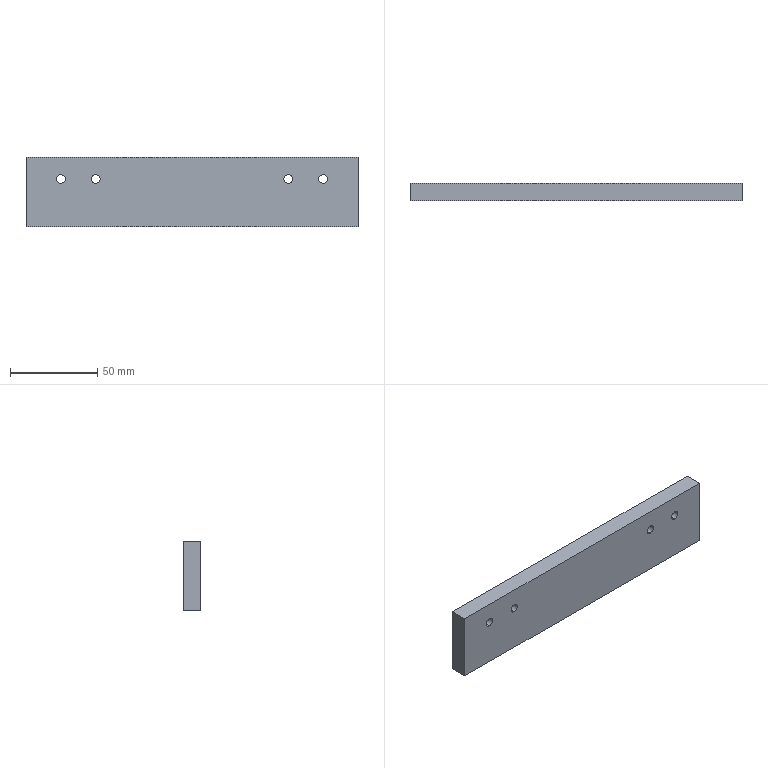Component | SolidWorks | SYM0671-81-101-1_SYM0671-81-108-1 | 1 solid | 14 faces | box 190 x 10 x 40 mm | volume 75215 mm3 | cylinder 8 | plane 6 | commonest cylinder face diameters 5 x8 | material AISI 304
build123d program:
from build123d import *

# Parameters (mm, degrees)
SKETCH1_W           = 40
SKETCH1_H           = 190
BOSS_EXTRUDE1_DEPTH = 10
M6_TAPPED_HOLE1_D   = 5


with BuildPart() as part:
    # Sketch1 → Boss-Extrude1 (new body)
    with BuildSketch(Plane.XY):
        Rectangle(SKETCH1_W, SKETCH1_H)
    extrude(amount=BOSS_EXTRUDE1_DEPTH)

    # M6 Tapped Hole1 (through all)
    with Locations(Plane.XY.offset(10)):
        with Locations((-7.5, -55), (-7.5, -75), (-7.5, 55), (-7.5, 75)):
            Hole(M6_TAPPED_HOLE1_D / 2)


solid = part.part

# Placed as in the assembly
solid = solid.moved(Location((61.751, -187.857, 280.518), (90, 0, -90)))
STEP:
#1=COLOUR_RGB('',0.7922,0.8196,0.9333);
#2=FILL_AREA_STYLE_COLOUR('',#1);
#3=FILL_AREA_STYLE('',(#2));
#4=SURFACE_STYLE_FILL_AREA(#3);
#5=SURFACE_SIDE_STYLE('',(#4));
#6=SURFACE_STYLE_USAGE(.BOTH.,#5);
#7=PRESENTATION_STYLE_ASSIGNMENT((#6));
#8=CARTESIAN_POINT('',(0.2658,-7.396,11.438));
#9=VERTEX_POINT('',#8);
#10=CARTESIAN_POINT('',(0.2658,-7.396,11.241));
#11=VERTEX_POINT('',#10);
#12=CARTESIAN_POINT('',(0.2658,-7.396,11.339));
#13=DIRECTION('',(0.,-1.,0.));
#14=DIRECTION('',(0.,0.,-1.));
#15=AXIS2_PLACEMENT_3D('',#12,#13,#14);
#16=CIRCLE('',#15,0.09843);
#17=EDGE_CURVE('',#9,#11,#16,.T.);
#18=ORIENTED_EDGE('',*,*,#17,.F.);
#19=CARTESIAN_POINT('',(0.2658,-7.79,11.438));
#20=VERTEX_POINT('',#19);
#21=CARTESIAN_POINT('',(0.2658,-7.79,11.438));
#22=DIRECTION('',(0.,-1.,0.));
#23=VECTOR('',#22,39.37);
#24=LINE('',#21,#23);
#25=EDGE_CURVE('',#9,#20,#24,.T.);
#26=ORIENTED_EDGE('',*,*,#25,.T.);
#27=CARTESIAN_POINT('',(0.2658,-7.79,11.241));
#28=VERTEX_POINT('',#27);
#29=CARTESIAN_POINT('',(0.2658,-7.79,11.339));
#30=DIRECTION('',(0.,-1.,0.));
#31=DIRECTION('',(0.,0.,-1.));
#32=AXIS2_PLACEMENT_3D('',#29,#30,#31);
#33=CIRCLE('',#32,0.09843);
#34=EDGE_CURVE('',#20,#28,#33,.T.);
#35=ORIENTED_EDGE('',*,*,#34,.T.);
#36=CARTESIAN_POINT('',(0.2658,-7.79,11.241));
#37=DIRECTION('',(0.,-1.,0.));
#38=VECTOR('',#37,39.37);
#39=LINE('',#36,#38);
#40=EDGE_CURVE('',#11,#28,#39,.T.);
#41=ORIENTED_EDGE('',*,*,#40,.F.);
#42=EDGE_LOOP('',(#18,#26,#35,#41));
#43=FACE_OUTER_BOUND('',#42,.T.);
#44=CARTESIAN_POINT('',(0.2658,-7.79,11.339));
#45=DIRECTION('',(0.,-1.,0.));
#46=DIRECTION('',(0.,0.,-1.));
#47=AXIS2_PLACEMENT_3D('',#44,#45,#46);
#48=CYLINDRICAL_SURFACE('',#47,0.09843);
#49=ADVANCED_FACE('',(#43),#48,.F.);
#50=CARTESIAN_POINT('',(-0.5216,-7.396,11.438));
#51=VERTEX_POINT('',#50);
#52=CARTESIAN_POINT('',(-0.5216,-7.396,11.241));
#53=VERTEX_POINT('',#52);
#54=CARTESIAN_POINT('',(-0.5216,-7.396,11.339));
#55=DIRECTION('',(0.,-1.,0.));
#56=DIRECTION('',(0.,0.,-1.));
#57=AXIS2_PLACEMENT_3D('',#54,#55,#56);
#58=CIRCLE('',#57,0.09843);
#59=EDGE_CURVE('',#51,#53,#58,.T.);
#60=ORIENTED_EDGE('',*,*,#59,.F.);
#61=CARTESIAN_POINT('',(-0.5216,-7.79,11.438));
#62=VERTEX_POINT('',#61);
#63=CARTESIAN_POINT('',(-0.5216,-7.79,11.438));
#64=DIRECTION('',(0.,-1.,0.));
#65=VECTOR('',#64,39.37);
#66=LINE('',#63,#65);
#67=EDGE_CURVE('',#51,#62,#66,.T.);
#68=ORIENTED_EDGE('',*,*,#67,.T.);
#69=CARTESIAN_POINT('',(-0.5216,-7.79,11.241));
#70=VERTEX_POINT('',#69);
#71=CARTESIAN_POINT('',(-0.5216,-7.79,11.339));
#72=DIRECTION('',(0.,-1.,0.));
#73=DIRECTION('',(0.,0.,-1.));
#74=AXIS2_PLACEMENT_3D('',#71,#72,#73);
#75=CIRCLE('',#74,0.09843);
#76=EDGE_CURVE('',#62,#70,#75,.T.);
#77=ORIENTED_EDGE('',*,*,#76,.T.);
#78=CARTESIAN_POINT('',(-0.5216,-7.79,11.241));
#79=DIRECTION('',(0.,-1.,0.));
#80=VECTOR('',#79,39.37);
#81=LINE('',#78,#80);
#82=EDGE_CURVE('',#53,#70,#81,.T.);
#83=ORIENTED_EDGE('',*,*,#82,.F.);
#84=EDGE_LOOP('',(#60,#68,#77,#83));
#85=FACE_OUTER_BOUND('',#84,.T.);
#86=CARTESIAN_POINT('',(-0.5216,-7.79,11.339));
#87=DIRECTION('',(0.,-1.,0.));
#88=DIRECTION('',(0.,0.,-1.));
#89=AXIS2_PLACEMENT_3D('',#86,#87,#88);
#90=CYLINDRICAL_SURFACE('',#89,0.09843);
#91=ADVANCED_FACE('',(#85),#90,.F.);
#92=CARTESIAN_POINT('',(4.597,-7.396,11.438));
#93=VERTEX_POINT('',#92);
#94=CARTESIAN_POINT('',(4.597,-7.396,11.241));
#95=VERTEX_POINT('',#94);
#96=CARTESIAN_POINT('',(4.597,-7.396,11.339));
#97=DIRECTION('',(0.,-1.,0.));
#98=DIRECTION('',(0.,0.,-1.));
#99=AXIS2_PLACEMENT_3D('',#96,#97,#98);
#100=CIRCLE('',#99,0.09843);
#101=EDGE_CURVE('',#93,#95,#100,.T.);
#102=ORIENTED_EDGE('',*,*,#101,.F.);
#103=CARTESIAN_POINT('',(4.597,-7.79,11.438));
#104=VERTEX_POINT('',#103);
#105=CARTESIAN_POINT('',(4.597,-7.79,11.438));
#106=DIRECTION('',(0.,-1.,0.));
#107=VECTOR('',#106,39.37);
#108=LINE('',#105,#107);
#109=EDGE_CURVE('',#93,#104,#108,.T.);
#110=ORIENTED_EDGE('',*,*,#109,.T.);
#111=CARTESIAN_POINT('',(4.597,-7.79,11.241));
#112=VERTEX_POINT('',#111);
#113=CARTESIAN_POINT('',(4.597,-7.79,11.339));
#114=DIRECTION('',(0.,-1.,0.));
#115=DIRECTION('',(0.,0.,-1.));
#116=AXIS2_PLACEMENT_3D('',#113,#114,#115);
#117=CIRCLE('',#116,0.09843);
#118=EDGE_CURVE('',#104,#112,#117,.T.);
#119=ORIENTED_EDGE('',*,*,#118,.T.);
#120=CARTESIAN_POINT('',(4.597,-7.79,11.241));
#121=DIRECTION('',(0.,-1.,0.));
#122=VECTOR('',#121,39.37);
#123=LINE('',#120,#122);
#124=EDGE_CURVE('',#95,#112,#123,.T.);
#125=ORIENTED_EDGE('',*,*,#124,.F.);
#126=EDGE_LOOP('',(#102,#110,#119,#125));
#127=FACE_OUTER_BOUND('',#126,.T.);
#128=CARTESIAN_POINT('',(4.597,-7.79,11.339));
#129=DIRECTION('',(0.,-1.,0.));
#130=DIRECTION('',(0.,0.,-1.));
#131=AXIS2_PLACEMENT_3D('',#128,#129,#130);
#132=CYLINDRICAL_SURFACE('',#131,0.09843);
#133=ADVANCED_FACE('',(#127),#132,.F.);
#134=CARTESIAN_POINT('',(5.384,-7.396,11.438));
#135=VERTEX_POINT('',#134);
#136=CARTESIAN_POINT('',(5.384,-7.396,11.241));
#137=VERTEX_POINT('',#136);
#138=CARTESIAN_POINT('',(5.384,-7.396,11.339));
#139=DIRECTION('',(0.,-1.,0.));
#140=DIRECTION('',(0.,0.,-1.));
#141=AXIS2_PLACEMENT_3D('',#138,#139,#140);
#142=CIRCLE('',#141,0.09843);
#143=EDGE_CURVE('',#135,#137,#142,.T.);
#144=ORIENTED_EDGE('',*,*,#143,.F.);
#145=CARTESIAN_POINT('',(5.384,-7.79,11.438));
#146=VERTEX_POINT('',#145);
#147=CARTESIAN_POINT('',(5.384,-7.79,11.438));
#148=DIRECTION('',(0.,-1.,0.));
#149=VECTOR('',#148,39.37);
#150=LINE('',#147,#149);
#151=EDGE_CURVE('',#135,#146,#150,.T.);
#152=ORIENTED_EDGE('',*,*,#151,.T.);
#153=CARTESIAN_POINT('',(5.384,-7.79,11.241));
#154=VERTEX_POINT('',#153);
#155=CARTESIAN_POINT('',(5.384,-7.79,11.339));
#156=DIRECTION('',(0.,-1.,0.));
#157=DIRECTION('',(0.,0.,-1.));
#158=AXIS2_PLACEMENT_3D('',#155,#156,#157);
#159=CIRCLE('',#158,0.09843);
#160=EDGE_CURVE('',#146,#154,#159,.T.);
#161=ORIENTED_EDGE('',*,*,#160,.T.);
#162=CARTESIAN_POINT('',(5.384,-7.79,11.241));
#163=DIRECTION('',(0.,-1.,0.));
#164=VECTOR('',#163,39.37);
#165=LINE('',#162,#164);
#166=EDGE_CURVE('',#137,#154,#165,.T.);
#167=ORIENTED_EDGE('',*,*,#166,.F.);
#168=EDGE_LOOP('',(#144,#152,#161,#167));
#169=FACE_OUTER_BOUND('',#168,.T.);
#170=CARTESIAN_POINT('',(5.384,-7.79,11.339));
#171=DIRECTION('',(0.,-1.,0.));
#172=DIRECTION('',(0.,0.,-1.));
#173=AXIS2_PLACEMENT_3D('',#170,#171,#172);
#174=CYLINDRICAL_SURFACE('',#173,0.09843);
#175=ADVANCED_FACE('',(#169),#174,.F.);
#176=CARTESIAN_POINT('',(-1.309,-7.396,10.257));
#177=VERTEX_POINT('',#176);
#178=CARTESIAN_POINT('',(6.171,-7.396,10.257));
#179=VERTEX_POINT('',#178);
#180=CARTESIAN_POINT('',(6.171,-7.396,10.257));
#181=DIRECTION('',(1.,0.,-0.));
#182=VECTOR('',#181,39.37);
#183=LINE('',#180,#182);
#184=EDGE_CURVE('',#177,#179,#183,.T.);
#185=ORIENTED_EDGE('',*,*,#184,.T.);
#186=CARTESIAN_POINT('',(6.171,-7.79,10.257));
#187=VERTEX_POINT('',#186);
#188=CARTESIAN_POINT('',(6.171,-7.79,10.257));
#189=DIRECTION('',(-0.,1.,-0.));
#190=VECTOR('',#189,39.37);
#191=LINE('',#188,#190);
#192=EDGE_CURVE('',#187,#179,#191,.T.);
#193=ORIENTED_EDGE('',*,*,#192,.F.);
#194=CARTESIAN_POINT('',(-1.309,-7.79,10.257));
#195=VERTEX_POINT('',#194);
#196=CARTESIAN_POINT('',(6.171,-7.79,10.257));
#197=DIRECTION('',(1.,0.,-0.));
#198=VECTOR('',#197,39.37);
#199=LINE('',#196,#198);
#200=EDGE_CURVE('',#195,#187,#199,.T.);
#201=ORIENTED_EDGE('',*,*,#200,.F.);
#202=CARTESIAN_POINT('',(-1.309,-7.79,10.257));
#203=DIRECTION('',(-0.,1.,-0.));
#204=VECTOR('',#203,39.37);
#205=LINE('',#202,#204);
#206=EDGE_CURVE('',#195,#177,#205,.T.);
#207=ORIENTED_EDGE('',*,*,#206,.T.);
#208=EDGE_LOOP('',(#185,#193,#201,#207));
#209=FACE_OUTER_BOUND('',#208,.T.);
#210=CARTESIAN_POINT('',(6.171,-7.79,10.257));
#211=DIRECTION('',(0.,0.,1.));
#212=DIRECTION('',(-1.,-0.,0.));
#213=AXIS2_PLACEMENT_3D('',#210,#211,#212);
#214=PLANE('',#213);
#215=ADVANCED_FACE('',(#209),#214,.F.);
#216=CARTESIAN_POINT('',(6.171,-7.396,11.831));
#217=VERTEX_POINT('',#216);
#218=CARTESIAN_POINT('',(6.171,-7.396,11.831));
#219=DIRECTION('',(0.,0.,1.));
#220=VECTOR('',#219,39.37);
#221=LINE('',#218,#220);
#222=EDGE_CURVE('',#179,#217,#221,.T.);
#223=ORIENTED_EDGE('',*,*,#222,.T.);
#224=CARTESIAN_POINT('',(6.171,-7.79,11.831));
#225=VERTEX_POINT('',#224);
#226=CARTESIAN_POINT('',(6.171,-7.79,11.831));
#227=DIRECTION('',(-0.,1.,-0.));
#228=VECTOR('',#227,39.37);
#229=LINE('',#226,#228);
#230=EDGE_CURVE('',#225,#217,#229,.T.);
#231=ORIENTED_EDGE('',*,*,#230,.F.);
#232=CARTESIAN_POINT('',(6.171,-7.79,11.831));
#233=DIRECTION('',(0.,0.,1.));
#234=VECTOR('',#233,39.37);
#235=LINE('',#232,#234);
#236=EDGE_CURVE('',#187,#225,#235,.T.);
#237=ORIENTED_EDGE('',*,*,#236,.F.);
#238=ORIENTED_EDGE('',*,*,#192,.T.);
#239=EDGE_LOOP('',(#223,#231,#237,#238));
#240=FACE_OUTER_BOUND('',#239,.T.);
#241=CARTESIAN_POINT('',(6.171,-7.79,11.831));
#242=DIRECTION('',(-1.,-0.,0.));
#243=DIRECTION('',(-0.,1.,-0.));
#244=AXIS2_PLACEMENT_3D('',#241,#242,#243);
#245=PLANE('',#244);
#246=ADVANCED_FACE('',(#240),#245,.F.);
#247=CARTESIAN_POINT('',(-1.309,-7.396,11.831));
#248=VERTEX_POINT('',#247);
#249=CARTESIAN_POINT('',(6.171,-7.396,11.831));
#250=DIRECTION('',(-1.,-0.,0.));
#251=VECTOR('',#250,39.37);
#252=LINE('',#249,#251);
#253=EDGE_CURVE('',#217,#248,#252,.T.);
#254=ORIENTED_EDGE('',*,*,#253,.T.);
#255=CARTESIAN_POINT('',(-1.309,-7.79,11.831));
#256=VERTEX_POINT('',#255);
#257=CARTESIAN_POINT('',(-1.309,-7.79,11.831));
#258=DIRECTION('',(-0.,1.,-0.));
#259=VECTOR('',#258,39.37);
#260=LINE('',#257,#259);
#261=EDGE_CURVE('',#256,#248,#260,.T.);
#262=ORIENTED_EDGE('',*,*,#261,.F.);
#263=CARTESIAN_POINT('',(6.171,-7.79,11.831));
#264=DIRECTION('',(-1.,-0.,0.));
#265=VECTOR('',#264,39.37);
#266=LINE('',#263,#265);
#267=EDGE_CURVE('',#225,#256,#266,.T.);
#268=ORIENTED_EDGE('',*,*,#267,.F.);
#269=ORIENTED_EDGE('',*,*,#230,.T.);
#270=EDGE_LOOP('',(#254,#262,#268,#269));
#271=FACE_OUTER_BOUND('',#270,.T.);
#272=CARTESIAN_POINT('',(6.171,-7.79,11.831));
#273=DIRECTION('',(-0.,-0.,-1.));
#274=DIRECTION('',(1.,0.,-0.));
#275=AXIS2_PLACEMENT_3D('',#272,#273,#274);
#276=PLANE('',#275);
#277=ADVANCED_FACE('',(#271),#276,.F.);
#278=CARTESIAN_POINT('',(-1.309,-7.396,11.831));
#279=DIRECTION('',(-0.,-0.,-1.));
#280=VECTOR('',#279,39.37);
#281=LINE('',#278,#280);
#282=EDGE_CURVE('',#248,#177,#281,.T.);
#283=ORIENTED_EDGE('',*,*,#282,.T.);
#284=ORIENTED_EDGE('',*,*,#206,.F.);
#285=CARTESIAN_POINT('',(-1.309,-7.79,11.831));
#286=DIRECTION('',(-0.,-0.,-1.));
#287=VECTOR('',#286,39.37);
#288=LINE('',#285,#287);
#289=EDGE_CURVE('',#256,#195,#288,.T.);
#290=ORIENTED_EDGE('',*,*,#289,.F.);
#291=ORIENTED_EDGE('',*,*,#261,.T.);
#292=EDGE_LOOP('',(#283,#284,#290,#291));
#293=FACE_OUTER_BOUND('',#292,.T.);
#294=CARTESIAN_POINT('',(-1.309,-7.79,11.831));
#295=DIRECTION('',(1.,0.,-0.));
#296=DIRECTION('',(0.,-1.,0.));
#297=AXIS2_PLACEMENT_3D('',#294,#295,#296);
#298=PLANE('',#297);
#299=ADVANCED_FACE('',(#293),#298,.F.);
#300=CARTESIAN_POINT('',(0.2658,-7.79,11.339));
#301=DIRECTION('',(0.,-1.,0.));
#302=DIRECTION('',(0.,0.,-1.));
#303=AXIS2_PLACEMENT_3D('',#300,#301,#302);
#304=CIRCLE('',#303,0.09843);
#305=EDGE_CURVE('',#28,#20,#304,.T.);
#306=ORIENTED_EDGE('',*,*,#305,.F.);
#307=ORIENTED_EDGE('',*,*,#34,.F.);
#308=EDGE_LOOP('',(#306,#307));
#309=FACE_BOUND('',#308,.T.);
#310=CARTESIAN_POINT('',(-0.5216,-7.79,11.339));
#311=DIRECTION('',(0.,-1.,0.));
#312=DIRECTION('',(0.,0.,-1.));
#313=AXIS2_PLACEMENT_3D('',#310,#311,#312);
#314=CIRCLE('',#313,0.09843);
#315=EDGE_CURVE('',#70,#62,#314,.T.);
#316=ORIENTED_EDGE('',*,*,#315,.F.);
#317=ORIENTED_EDGE('',*,*,#76,.F.);
#318=EDGE_LOOP('',(#316,#317));
#319=FACE_BOUND('',#318,.T.);
#320=CARTESIAN_POINT('',(4.597,-7.79,11.339));
#321=DIRECTION('',(0.,-1.,0.));
#322=DIRECTION('',(0.,0.,-1.));
#323=AXIS2_PLACEMENT_3D('',#320,#321,#322);
#324=CIRCLE('',#323,0.09843);
#325=EDGE_CURVE('',#112,#104,#324,.T.);
#326=ORIENTED_EDGE('',*,*,#325,.F.);
#327=ORIENTED_EDGE('',*,*,#118,.F.);
#328=EDGE_LOOP('',(#326,#327));
#329=FACE_BOUND('',#328,.T.);
#330=CARTESIAN_POINT('',(5.384,-7.79,11.339));
#331=DIRECTION('',(0.,-1.,0.));
#332=DIRECTION('',(0.,0.,-1.));
#333=AXIS2_PLACEMENT_3D('',#330,#331,#332);
#334=CIRCLE('',#333,0.09843);
#335=EDGE_CURVE('',#154,#146,#334,.T.);
#336=ORIENTED_EDGE('',*,*,#335,.F.);
#337=ORIENTED_EDGE('',*,*,#160,.F.);
#338=EDGE_LOOP('',(#336,#337));
#339=FACE_BOUND('',#338,.T.);
#340=ORIENTED_EDGE('',*,*,#200,.T.);
#341=ORIENTED_EDGE('',*,*,#236,.T.);
#342=ORIENTED_EDGE('',*,*,#267,.T.);
#343=ORIENTED_EDGE('',*,*,#289,.T.);
#344=EDGE_LOOP('',(#340,#341,#342,#343));
#345=FACE_OUTER_BOUND('',#344,.T.);
#346=CARTESIAN_POINT('',(-1.309,-7.79,10.257));
#347=DIRECTION('',(0.,-1.,0.));
#348=DIRECTION('',(-0.,-0.,-1.));
#349=AXIS2_PLACEMENT_3D('',#346,#347,#348);
#350=PLANE('',#349);
#351=ADVANCED_FACE('',(#309,#319,#329,#339,#345),#350,.T.);
#352=CARTESIAN_POINT('',(0.2658,-7.396,11.339));
#353=DIRECTION('',(0.,-1.,0.));
#354=DIRECTION('',(0.,0.,-1.));
#355=AXIS2_PLACEMENT_3D('',#352,#353,#354);
#356=CIRCLE('',#355,0.09843);
#357=EDGE_CURVE('',#11,#9,#356,.T.);
#358=ORIENTED_EDGE('',*,*,#357,.T.);
#359=ORIENTED_EDGE('',*,*,#17,.T.);
#360=EDGE_LOOP('',(#358,#359));
#361=FACE_BOUND('',#360,.T.);
#362=CARTESIAN_POINT('',(-0.5216,-7.396,11.339));
#363=DIRECTION('',(0.,-1.,0.));
#364=DIRECTION('',(0.,0.,-1.));
#365=AXIS2_PLACEMENT_3D('',#362,#363,#364);
#366=CIRCLE('',#365,0.09843);
#367=EDGE_CURVE('',#53,#51,#366,.T.);
#368=ORIENTED_EDGE('',*,*,#367,.T.);
#369=ORIENTED_EDGE('',*,*,#59,.T.);
#370=EDGE_LOOP('',(#368,#369));
#371=FACE_BOUND('',#370,.T.);
#372=CARTESIAN_POINT('',(4.597,-7.396,11.339));
#373=DIRECTION('',(0.,-1.,0.));
#374=DIRECTION('',(0.,0.,-1.));
#375=AXIS2_PLACEMENT_3D('',#372,#373,#374);
#376=CIRCLE('',#375,0.09843);
#377=EDGE_CURVE('',#95,#93,#376,.T.);
#378=ORIENTED_EDGE('',*,*,#377,.T.);
#379=ORIENTED_EDGE('',*,*,#101,.T.);
#380=EDGE_LOOP('',(#378,#379));
#381=FACE_BOUND('',#380,.T.);
#382=CARTESIAN_POINT('',(5.384,-7.396,11.339));
#383=DIRECTION('',(0.,-1.,0.));
#384=DIRECTION('',(0.,0.,-1.));
#385=AXIS2_PLACEMENT_3D('',#382,#383,#384);
#386=CIRCLE('',#385,0.09843);
#387=EDGE_CURVE('',#137,#135,#386,.T.);
#388=ORIENTED_EDGE('',*,*,#387,.T.);
#389=ORIENTED_EDGE('',*,*,#143,.T.);
#390=EDGE_LOOP('',(#388,#389));
#391=FACE_BOUND('',#390,.T.);
#392=ORIENTED_EDGE('',*,*,#184,.F.);
#393=ORIENTED_EDGE('',*,*,#282,.F.);
#394=ORIENTED_EDGE('',*,*,#253,.F.);
#395=ORIENTED_EDGE('',*,*,#222,.F.);
#396=EDGE_LOOP('',(#392,#393,#394,#395));
#397=FACE_OUTER_BOUND('',#396,.T.);
#398=CARTESIAN_POINT('',(-1.309,-7.396,10.257));
#399=DIRECTION('',(0.,-1.,0.));
#400=DIRECTION('',(-0.,-0.,-1.));
#401=AXIS2_PLACEMENT_3D('',#398,#399,#400);
#402=PLANE('',#401);
#403=ADVANCED_FACE('',(#361,#371,#381,#391,#397),#402,.F.);
#404=ORIENTED_EDGE('',*,*,#151,.F.);
#405=ORIENTED_EDGE('',*,*,#387,.F.);
#406=ORIENTED_EDGE('',*,*,#166,.T.);
#407=ORIENTED_EDGE('',*,*,#335,.T.);
#408=EDGE_LOOP('',(#404,#405,#406,#407));
#409=FACE_OUTER_BOUND('',#408,.T.);
#410=CARTESIAN_POINT('',(5.384,-7.79,11.339));
#411=DIRECTION('',(0.,-1.,0.));
#412=DIRECTION('',(0.,0.,-1.));
#413=AXIS2_PLACEMENT_3D('',#410,#411,#412);
#414=CYLINDRICAL_SURFACE('',#413,0.09843);
#415=ADVANCED_FACE('',(#409),#414,.F.);
#416=ORIENTED_EDGE('',*,*,#109,.F.);
#417=ORIENTED_EDGE('',*,*,#377,.F.);
#418=ORIENTED_EDGE('',*,*,#124,.T.);
#419=ORIENTED_EDGE('',*,*,#325,.T.);
#420=EDGE_LOOP('',(#416,#417,#418,#419));
#421=FACE_OUTER_BOUND('',#420,.T.);
#422=CARTESIAN_POINT('',(4.597,-7.79,11.339));
#423=DIRECTION('',(0.,-1.,0.));
#424=DIRECTION('',(0.,0.,-1.));
#425=AXIS2_PLACEMENT_3D('',#422,#423,#424);
#426=CYLINDRICAL_SURFACE('',#425,0.09843);
#427=ADVANCED_FACE('',(#421),#426,.F.);
#428=ORIENTED_EDGE('',*,*,#67,.F.);
#429=ORIENTED_EDGE('',*,*,#367,.F.);
#430=ORIENTED_EDGE('',*,*,#82,.T.);
#431=ORIENTED_EDGE('',*,*,#315,.T.);
#432=EDGE_LOOP('',(#428,#429,#430,#431));
#433=FACE_OUTER_BOUND('',#432,.T.);
#434=CARTESIAN_POINT('',(-0.5216,-7.79,11.339));
#435=DIRECTION('',(0.,-1.,0.));
#436=DIRECTION('',(0.,0.,-1.));
#437=AXIS2_PLACEMENT_3D('',#434,#435,#436);
#438=CYLINDRICAL_SURFACE('',#437,0.09843);
#439=ADVANCED_FACE('',(#433),#438,.F.);
#440=ORIENTED_EDGE('',*,*,#25,.F.);
#441=ORIENTED_EDGE('',*,*,#357,.F.);
#442=ORIENTED_EDGE('',*,*,#40,.T.);
#443=ORIENTED_EDGE('',*,*,#305,.T.);
#444=EDGE_LOOP('',(#440,#441,#442,#443));
#445=FACE_OUTER_BOUND('',#444,.T.);
#446=CARTESIAN_POINT('',(0.2658,-7.79,11.339));
#447=DIRECTION('',(0.,-1.,0.));
#448=DIRECTION('',(0.,0.,-1.));
#449=AXIS2_PLACEMENT_3D('',#446,#447,#448);
#450=CYLINDRICAL_SURFACE('',#449,0.09843);
#451=ADVANCED_FACE('',(#445),#450,.F.);
#452=CLOSED_SHELL('',(#49,#91,#133,#175,#215,#246,#277,#299,#351,#403,#415,#427,#439,#451));
#453=MANIFOLD_SOLID_BREP('',#452);
#454=STYLED_ITEM('',(#7),#453);
#455=PRESENTATION_LAYER_ASSIGNMENT('','',(#454));
#456=CARTESIAN_POINT('',(0.,0.,0.));
#457=DIRECTION('',(0.,0.,1.));
#458=DIRECTION('',(1.,0.,0.));
#459=AXIS2_PLACEMENT_3D('',#456,#457,#458);
#460=(LENGTH_UNIT()NAMED_UNIT(*)SI_UNIT($,.METRE.));
#461=LENGTH_MEASURE_WITH_UNIT(LENGTH_MEASURE(0.0254),#460);
#462=DIMENSIONAL_EXPONENTS(1.,0.,0.,0.,0.,0.,0.);
#463=(CONVERSION_BASED_UNIT('',#461)LENGTH_UNIT()NAMED_UNIT(#462));
#464=UNCERTAINTY_MEASURE_WITH_UNIT(LENGTH_MEASURE(0.00001),#463,'','');
#465=(NAMED_UNIT(*)PLANE_ANGLE_UNIT()SI_UNIT($,.RADIAN.));
#466=(NAMED_UNIT(*)SI_UNIT($,.STERADIAN.)SOLID_ANGLE_UNIT());
#467=(GEOMETRIC_REPRESENTATION_CONTEXT(3)GLOBAL_UNCERTAINTY_ASSIGNED_CONTEXT((#464))GLOBAL_UNIT_ASSIGNED_CONTEXT((#463,#465,#466))REPRESENTATION_CONTEXT('',''));
#468=ADVANCED_BREP_SHAPE_REPRESENTATION('',(#453,#459),#467);
#469=(LENGTH_UNIT()NAMED_UNIT(*)SI_UNIT($,.METRE.));
#470=LENGTH_MEASURE_WITH_UNIT(LENGTH_MEASURE(0.0254),#469);
#471=DIMENSIONAL_EXPONENTS(1.,0.,0.,0.,0.,0.,0.);
#472=(CONVERSION_BASED_UNIT('',#470)LENGTH_UNIT()NAMED_UNIT(#471));
#473=UNCERTAINTY_MEASURE_WITH_UNIT(LENGTH_MEASURE(0.00001),#472,'','');
#474=(NAMED_UNIT(*)PLANE_ANGLE_UNIT()SI_UNIT($,.RADIAN.));
#475=(NAMED_UNIT(*)SI_UNIT($,.STERADIAN.)SOLID_ANGLE_UNIT());
#476=(GEOMETRIC_REPRESENTATION_CONTEXT(3)GLOBAL_UNCERTAINTY_ASSIGNED_CONTEXT((#473))GLOBAL_UNIT_ASSIGNED_CONTEXT((#472,#474,#475))REPRESENTATION_CONTEXT('',''));
#477=MECHANICAL_DESIGN_GEOMETRIC_PRESENTATION_REPRESENTATION('',(#454),#476);